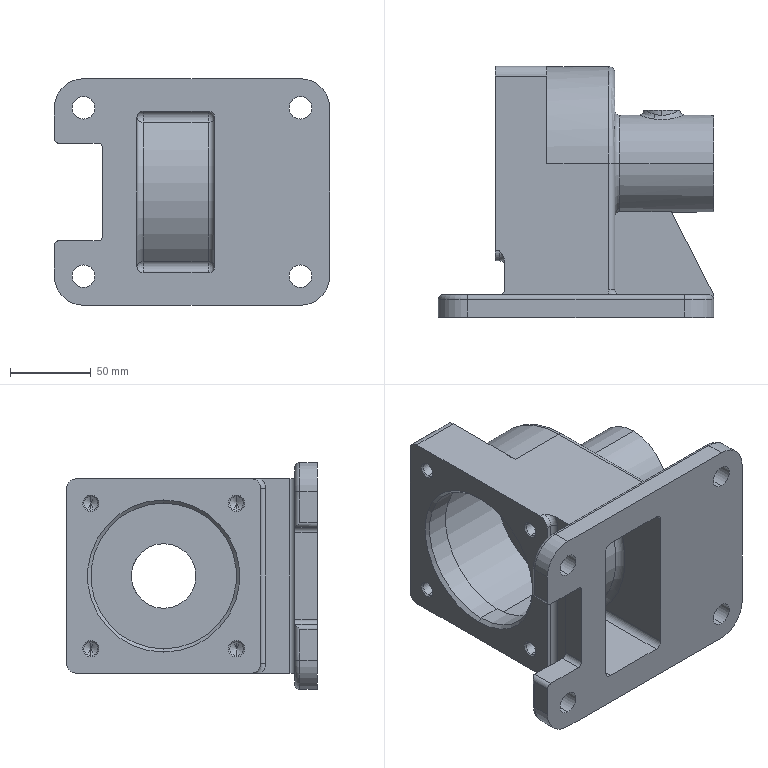Component | SolidWorks | Box151-1 | 1 solid | 144 faces | volume 885293 mm3 | cylinder 70 | plane 34 | cone 20 | torus 14 | sphere 4 | spline 2 | commonest cylinder face diameters 6 x15 28 x8 14 x8 8.5 x8 8 x8 36 x4 12 x4 22 x3